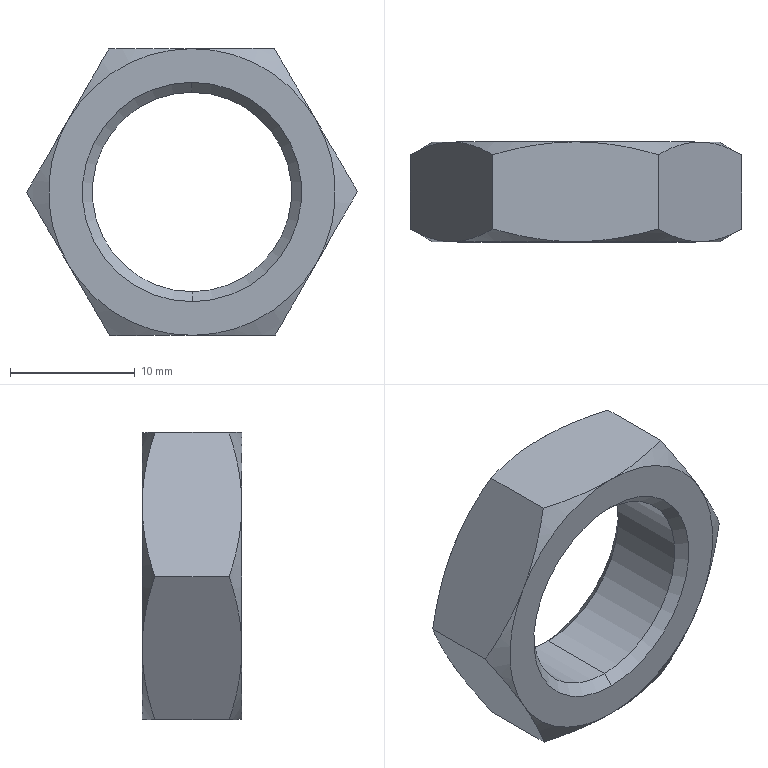Component | SolidWorks | NewCurveBenderSC63x40Cylinder-DoubleWheel-1_NewTypeCurveBenderM16x1_5-Nut-DoubleWheel-2 | 1 solid | 26 faces | box 26.56 x 8 x 23.05 mm | volume 1997 mm3 | cone 16 | plane 8 | cylinder 2 | commonest cylinder face diameters 16 x2
STEP:
#1=COLOUR_RGB('',0.7922,0.8196,0.9333);
#2=FILL_AREA_STYLE_COLOUR('',#1);
#3=FILL_AREA_STYLE('',(#2));
#4=SURFACE_STYLE_FILL_AREA(#3);
#5=SURFACE_SIDE_STYLE('',(#4));
#6=SURFACE_STYLE_USAGE(.BOTH.,#5);
#7=PRESENTATION_STYLE_ASSIGNMENT((#6));
#8=CARTESIAN_POINT('',(1.967,-10.583,0.315));
#9=VERTEX_POINT('',#8);
#10=CARTESIAN_POINT('',(1.97,-10.583,-0.315));
#11=VERTEX_POINT('',#10);
#12=CARTESIAN_POINT('',(1.969,-10.583,0.));
#13=DIRECTION('',(0.,-1.,-0.));
#14=DIRECTION('',(0.003512,0.,-1.));
#15=AXIS2_PLACEMENT_3D('',#12,#13,#14);
#16=CIRCLE('',#15,0.315);
#17=EDGE_CURVE('',#9,#11,#16,.T.);
#18=ORIENTED_EDGE('',*,*,#17,.T.);
#19=CARTESIAN_POINT('',(1.97,-10.551,-0.3465));
#20=VERTEX_POINT('',#19);
#21=CARTESIAN_POINT('',(1.97,-10.551,-0.3465));
#22=DIRECTION('',(0.002484,0.7071,-0.7071));
#23=VECTOR('',#22,39.37);
#24=LINE('',#21,#23);
#25=EDGE_CURVE('',#11,#20,#24,.T.);
#26=ORIENTED_EDGE('',*,*,#25,.T.);
#27=CARTESIAN_POINT('',(1.967,-10.551,0.3465));
#28=VERTEX_POINT('',#27);
#29=CARTESIAN_POINT('',(1.969,-10.551,0.));
#30=DIRECTION('',(0.,-1.,-0.));
#31=DIRECTION('',(0.003512,0.,-1.));
#32=AXIS2_PLACEMENT_3D('',#29,#30,#31);
#33=CIRCLE('',#32,0.3465);
#34=EDGE_CURVE('',#28,#20,#33,.T.);
#35=ORIENTED_EDGE('',*,*,#34,.F.);
#36=CARTESIAN_POINT('',(1.967,-10.551,0.3465));
#37=DIRECTION('',(-0.002484,0.7071,0.7071));
#38=VECTOR('',#37,39.37);
#39=LINE('',#36,#38);
#40=EDGE_CURVE('',#9,#28,#39,.T.);
#41=ORIENTED_EDGE('',*,*,#40,.F.);
#42=EDGE_LOOP('',(#18,#26,#35,#41));
#43=FACE_OUTER_BOUND('',#42,.T.);
#44=CARTESIAN_POINT('',(1.969,-10.551,0.));
#45=DIRECTION('',(-0.,1.,0.));
#46=DIRECTION('',(-0.003512,0.,1.));
#47=AXIS2_PLACEMENT_3D('',#44,#45,#46);
#48=CONICAL_SURFACE('',#47,0.3465,0.7854);
#49=ADVANCED_FACE('',(#43),#48,.F.);
#50=ORIENTED_EDGE('',*,*,#17,.F.);
#51=CARTESIAN_POINT('',(1.967,-10.835,0.315));
#52=VERTEX_POINT('',#51);
#53=CARTESIAN_POINT('',(1.967,-10.551,0.315));
#54=DIRECTION('',(0.,-1.,-0.));
#55=VECTOR('',#54,39.37);
#56=LINE('',#53,#55);
#57=EDGE_CURVE('',#9,#52,#56,.T.);
#58=ORIENTED_EDGE('',*,*,#57,.T.);
#59=CARTESIAN_POINT('',(1.97,-10.835,-0.315));
#60=VERTEX_POINT('',#59);
#61=CARTESIAN_POINT('',(1.969,-10.835,0.));
#62=DIRECTION('',(0.,-1.,-0.));
#63=DIRECTION('',(0.003512,0.,-1.));
#64=AXIS2_PLACEMENT_3D('',#61,#62,#63);
#65=CIRCLE('',#64,0.315);
#66=EDGE_CURVE('',#52,#60,#65,.T.);
#67=ORIENTED_EDGE('',*,*,#66,.T.);
#68=CARTESIAN_POINT('',(1.97,-10.551,-0.315));
#69=DIRECTION('',(0.,-1.,-0.));
#70=VECTOR('',#69,39.37);
#71=LINE('',#68,#70);
#72=EDGE_CURVE('',#11,#60,#71,.T.);
#73=ORIENTED_EDGE('',*,*,#72,.F.);
#74=EDGE_LOOP('',(#50,#58,#67,#73));
#75=FACE_OUTER_BOUND('',#74,.T.);
#76=CARTESIAN_POINT('',(1.969,-10.551,0.));
#77=DIRECTION('',(0.,-1.,-0.));
#78=DIRECTION('',(0.003512,0.,-1.));
#79=AXIS2_PLACEMENT_3D('',#76,#77,#78);
#80=CYLINDRICAL_SURFACE('',#79,0.315);
#81=ADVANCED_FACE('',(#75),#80,.F.);
#82=ORIENTED_EDGE('',*,*,#66,.F.);
#83=CARTESIAN_POINT('',(1.967,-10.866,0.3465));
#84=VERTEX_POINT('',#83);
#85=CARTESIAN_POINT('',(1.967,-10.835,0.315));
#86=DIRECTION('',(-0.002484,-0.7071,0.7071));
#87=VECTOR('',#86,39.37);
#88=LINE('',#85,#87);
#89=EDGE_CURVE('',#52,#84,#88,.T.);
#90=ORIENTED_EDGE('',*,*,#89,.T.);
#91=CARTESIAN_POINT('',(1.97,-10.866,-0.3465));
#92=VERTEX_POINT('',#91);
#93=CARTESIAN_POINT('',(1.969,-10.866,0.));
#94=DIRECTION('',(0.,-1.,-0.));
#95=DIRECTION('',(0.003512,0.,-1.));
#96=AXIS2_PLACEMENT_3D('',#93,#94,#95);
#97=CIRCLE('',#96,0.3465);
#98=EDGE_CURVE('',#84,#92,#97,.T.);
#99=ORIENTED_EDGE('',*,*,#98,.T.);
#100=CARTESIAN_POINT('',(1.97,-10.835,-0.315));
#101=DIRECTION('',(0.002484,-0.7071,-0.7071));
#102=VECTOR('',#101,39.37);
#103=LINE('',#100,#102);
#104=EDGE_CURVE('',#60,#92,#103,.T.);
#105=ORIENTED_EDGE('',*,*,#104,.F.);
#106=EDGE_LOOP('',(#82,#90,#99,#105));
#107=FACE_OUTER_BOUND('',#106,.T.);
#108=CARTESIAN_POINT('',(1.969,-10.835,0.));
#109=DIRECTION('',(0.,-1.,-0.));
#110=DIRECTION('',(0.003512,0.,-1.));
#111=AXIS2_PLACEMENT_3D('',#108,#109,#110);
#112=CONICAL_SURFACE('',#111,0.315,0.7854);
#113=ADVANCED_FACE('',(#107),#112,.F.);
#114=CARTESIAN_POINT('',(1.967,-10.866,0.4528));
#115=VERTEX_POINT('',#114);
#116=CARTESIAN_POINT('',(1.706,-10.826,0.4518));
#117=VERTEX_POINT('',#116);
#118=CARTESIAN_POINT('',(1.967,-10.866,0.4528));
#119=CARTESIAN_POINT('',(1.923,-10.866,0.4526));
#120=CARTESIAN_POINT('',(1.879,-10.862,0.4524));
#121=CARTESIAN_POINT('',(1.792,-10.848,0.4521));
#122=CARTESIAN_POINT('',(1.748,-10.838,0.452));
#123=CARTESIAN_POINT('',(1.706,-10.826,0.4518));
#124=B_SPLINE_CURVE_WITH_KNOTS('',3,(#118,#119,#120,#121,#122,#123),.UNSPECIFIED.,.F.,.F.,(4,2,4),(0.03588,0.03924,0.0426),.UNSPECIFIED.);
#125=EDGE_CURVE('',#115,#117,#124,.T.);
#126=ORIENTED_EDGE('',*,*,#125,.T.);
#127=CARTESIAN_POINT('',(1.576,-10.866,0.225));
#128=VERTEX_POINT('',#127);
#129=CARTESIAN_POINT('',(1.706,-10.826,0.4518));
#130=CARTESIAN_POINT('',(1.684,-10.838,0.4147));
#131=CARTESIAN_POINT('',(1.663,-10.848,0.3773));
#132=CARTESIAN_POINT('',(1.62,-10.862,0.3018));
#133=CARTESIAN_POINT('',(1.598,-10.866,0.2636));
#134=CARTESIAN_POINT('',(1.576,-10.866,0.225));
#135=B_SPLINE_CURVE_WITH_KNOTS('',3,(#129,#130,#131,#132,#133,#134),.UNSPECIFIED.,.F.,.F.,(4,2,4),(0.00000024,0.003359,0.006718),.UNSPECIFIED.);
#136=EDGE_CURVE('',#117,#128,#135,.T.);
#137=ORIENTED_EDGE('',*,*,#136,.T.);
#138=CARTESIAN_POINT('',(1.969,-10.866,0.));
#139=DIRECTION('',(0.,-1.,-0.));
#140=DIRECTION('',(0.003512,0.,-1.));
#141=AXIS2_PLACEMENT_3D('',#138,#139,#140);
#142=CIRCLE('',#141,0.4528);
#143=EDGE_CURVE('',#115,#128,#142,.T.);
#144=ORIENTED_EDGE('',*,*,#143,.F.);
#145=EDGE_LOOP('',(#126,#137,#144));
#146=FACE_OUTER_BOUND('',#145,.T.);
#147=CARTESIAN_POINT('',(1.969,-10.814,0.));
#148=DIRECTION('',(-0.,1.,0.));
#149=DIRECTION('',(-0.003512,0.,1.));
#150=AXIS2_PLACEMENT_3D('',#147,#148,#149);
#151=CONICAL_SURFACE('',#150,0.5433,1.047);
#152=ADVANCED_FACE('',(#146),#151,.T.);
#153=CARTESIAN_POINT('',(1.577,-10.866,-0.2278));
#154=VERTEX_POINT('',#153);
#155=CARTESIAN_POINT('',(1.969,-10.866,0.));
#156=DIRECTION('',(0.,-1.,-0.));
#157=DIRECTION('',(0.003512,0.,-1.));
#158=AXIS2_PLACEMENT_3D('',#155,#156,#157);
#159=CIRCLE('',#158,0.4528);
#160=EDGE_CURVE('',#128,#154,#159,.T.);
#161=ORIENTED_EDGE('',*,*,#160,.F.);
#162=CARTESIAN_POINT('',(1.446,-10.826,-0.001836));
#163=VERTEX_POINT('',#162);
#164=CARTESIAN_POINT('',(1.576,-10.866,0.225));
#165=CARTESIAN_POINT('',(1.565,-10.866,0.2057));
#166=CARTESIAN_POINT('',(1.554,-10.865,0.1864));
#167=CARTESIAN_POINT('',(1.532,-10.861,0.1482));
#168=CARTESIAN_POINT('',(1.521,-10.859,0.1292));
#169=CARTESIAN_POINT('',(1.488,-10.848,0.0725));
#170=CARTESIAN_POINT('',(1.467,-10.838,0.03518));
#171=CARTESIAN_POINT('',(1.446,-10.826,-0.001836));
#172=B_SPLINE_CURVE_WITH_KNOTS('',3,(#164,#165,#166,#167,#168,#169,#170,#171),.UNSPECIFIED.,.F.,.F.,(4,2,2,4),(0.006718,0.008392,0.01006,0.01341),.UNSPECIFIED.);
#173=EDGE_CURVE('',#128,#163,#172,.T.);
#174=ORIENTED_EDGE('',*,*,#173,.T.);
#175=CARTESIAN_POINT('',(1.446,-10.826,-0.001836));
#176=CARTESIAN_POINT('',(1.467,-10.838,-0.03879));
#177=CARTESIAN_POINT('',(1.489,-10.848,-0.07602));
#178=CARTESIAN_POINT('',(1.533,-10.862,-0.1513));
#179=CARTESIAN_POINT('',(1.555,-10.866,-0.1893));
#180=CARTESIAN_POINT('',(1.577,-10.866,-0.2278));
#181=B_SPLINE_CURVE_WITH_KNOTS('',3,(#175,#176,#177,#178,#179,#180),.UNSPECIFIED.,.F.,.F.,(4,2,4),(0.00000024,0.003359,0.006718),.UNSPECIFIED.);
#182=EDGE_CURVE('',#163,#154,#181,.T.);
#183=ORIENTED_EDGE('',*,*,#182,.T.);
#184=EDGE_LOOP('',(#161,#174,#183));
#185=FACE_OUTER_BOUND('',#184,.T.);
#186=CARTESIAN_POINT('',(1.969,-10.814,0.));
#187=DIRECTION('',(-0.,1.,0.));
#188=DIRECTION('',(-0.003512,0.,1.));
#189=AXIS2_PLACEMENT_3D('',#186,#187,#188);
#190=CONICAL_SURFACE('',#189,0.5433,1.047);
#191=ADVANCED_FACE('',(#185),#190,.T.);
#192=CARTESIAN_POINT('',(1.97,-10.866,-0.4528));
#193=VERTEX_POINT('',#192);
#194=CARTESIAN_POINT('',(1.969,-10.866,0.));
#195=DIRECTION('',(0.,-1.,-0.));
#196=DIRECTION('',(0.003512,0.,-1.));
#197=AXIS2_PLACEMENT_3D('',#194,#195,#196);
#198=CIRCLE('',#197,0.4528);
#199=EDGE_CURVE('',#154,#193,#198,.T.);
#200=ORIENTED_EDGE('',*,*,#199,.F.);
#201=CARTESIAN_POINT('',(1.709,-10.826,-0.4537));
#202=VERTEX_POINT('',#201);
#203=CARTESIAN_POINT('',(1.577,-10.866,-0.2278));
#204=CARTESIAN_POINT('',(1.588,-10.866,-0.2469));
#205=CARTESIAN_POINT('',(1.6,-10.865,-0.2662));
#206=CARTESIAN_POINT('',(1.622,-10.861,-0.3043));
#207=CARTESIAN_POINT('',(1.633,-10.859,-0.3232));
#208=CARTESIAN_POINT('',(1.666,-10.848,-0.3796));
#209=CARTESIAN_POINT('',(1.687,-10.838,-0.4168));
#210=CARTESIAN_POINT('',(1.709,-10.826,-0.4537));
#211=B_SPLINE_CURVE_WITH_KNOTS('',3,(#203,#204,#205,#206,#207,#208,#209,#210),.UNSPECIFIED.,.F.,.F.,(4,2,2,4),(0.006718,0.008392,0.01006,0.01341),.UNSPECIFIED.);
#212=EDGE_CURVE('',#154,#202,#211,.T.);
#213=ORIENTED_EDGE('',*,*,#212,.T.);
#214=CARTESIAN_POINT('',(1.709,-10.826,-0.4537));
#215=CARTESIAN_POINT('',(1.751,-10.838,-0.4535));
#216=CARTESIAN_POINT('',(1.795,-10.848,-0.4534));
#217=CARTESIAN_POINT('',(1.882,-10.862,-0.4531));
#218=CARTESIAN_POINT('',(1.926,-10.866,-0.4529));
#219=CARTESIAN_POINT('',(1.97,-10.866,-0.4528));
#220=B_SPLINE_CURVE_WITH_KNOTS('',3,(#214,#215,#216,#217,#218,#219),.UNSPECIFIED.,.F.,.F.,(4,2,4),(0.01189,0.01525,0.01861),.UNSPECIFIED.);
#221=EDGE_CURVE('',#202,#193,#220,.T.);
#222=ORIENTED_EDGE('',*,*,#221,.T.);
#223=EDGE_LOOP('',(#200,#213,#222));
#224=FACE_OUTER_BOUND('',#223,.T.);
#225=CARTESIAN_POINT('',(1.969,-10.814,0.));
#226=DIRECTION('',(-0.,1.,0.));
#227=DIRECTION('',(-0.003512,0.,1.));
#228=AXIS2_PLACEMENT_3D('',#225,#226,#227);
#229=CONICAL_SURFACE('',#228,0.5433,1.047);
#230=ADVANCED_FACE('',(#224),#229,.T.);
#231=CARTESIAN_POINT('',(2.36,-10.866,0.2278));
#232=VERTEX_POINT('',#231);
#233=CARTESIAN_POINT('',(2.228,-10.826,0.4537));
#234=VERTEX_POINT('',#233);
#235=CARTESIAN_POINT('',(2.36,-10.866,0.2278));
#236=CARTESIAN_POINT('',(2.349,-10.866,0.2469));
#237=CARTESIAN_POINT('',(2.337,-10.865,0.2662));
#238=CARTESIAN_POINT('',(2.315,-10.861,0.3043));
#239=CARTESIAN_POINT('',(2.304,-10.859,0.3232));
#240=CARTESIAN_POINT('',(2.271,-10.848,0.3796));
#241=CARTESIAN_POINT('',(2.25,-10.838,0.4168));
#242=CARTESIAN_POINT('',(2.228,-10.826,0.4537));
#243=B_SPLINE_CURVE_WITH_KNOTS('',3,(#235,#236,#237,#238,#239,#240,#241,#242),.UNSPECIFIED.,.F.,.F.,(4,2,2,4),(0.006718,0.008392,0.01006,0.01341),.UNSPECIFIED.);
#244=EDGE_CURVE('',#232,#234,#243,.T.);
#245=ORIENTED_EDGE('',*,*,#244,.T.);
#246=CARTESIAN_POINT('',(2.228,-10.826,0.4537));
#247=CARTESIAN_POINT('',(2.186,-10.838,0.4535));
#248=CARTESIAN_POINT('',(2.143,-10.848,0.4534));
#249=CARTESIAN_POINT('',(2.078,-10.859,0.4531));
#250=CARTESIAN_POINT('',(2.056,-10.861,0.4531));
#251=CARTESIAN_POINT('',(2.011,-10.865,0.4529));
#252=CARTESIAN_POINT('',(1.989,-10.866,0.4528));
#253=CARTESIAN_POINT('',(1.967,-10.866,0.4528));
#254=B_SPLINE_CURVE_WITH_KNOTS('',3,(#246,#247,#248,#249,#250,#251,#252,#253),.UNSPECIFIED.,.F.,.F.,(4,2,2,4),(0.02915,0.03251,0.03419,0.03588),.UNSPECIFIED.);
#255=EDGE_CURVE('',#234,#115,#254,.T.);
#256=ORIENTED_EDGE('',*,*,#255,.T.);
#257=CARTESIAN_POINT('',(1.969,-10.866,0.));
#258=DIRECTION('',(0.,-1.,-0.));
#259=DIRECTION('',(0.003512,0.,-1.));
#260=AXIS2_PLACEMENT_3D('',#257,#258,#259);
#261=CIRCLE('',#260,0.4528);
#262=EDGE_CURVE('',#232,#115,#261,.T.);
#263=ORIENTED_EDGE('',*,*,#262,.F.);
#264=EDGE_LOOP('',(#245,#256,#263));
#265=FACE_OUTER_BOUND('',#264,.T.);
#266=CARTESIAN_POINT('',(1.969,-10.814,0.));
#267=DIRECTION('',(-0.,1.,0.));
#268=DIRECTION('',(-0.003512,0.,1.));
#269=AXIS2_PLACEMENT_3D('',#266,#267,#268);
#270=CONICAL_SURFACE('',#269,0.5433,1.047);
#271=ADVANCED_FACE('',(#265),#270,.T.);
#272=CARTESIAN_POINT('',(2.361,-10.866,-0.225));
#273=VERTEX_POINT('',#272);
#274=CARTESIAN_POINT('',(1.969,-10.866,0.));
#275=DIRECTION('',(0.,-1.,-0.));
#276=DIRECTION('',(0.003512,0.,-1.));
#277=AXIS2_PLACEMENT_3D('',#274,#275,#276);
#278=CIRCLE('',#277,0.4528);
#279=EDGE_CURVE('',#193,#273,#278,.T.);
#280=ORIENTED_EDGE('',*,*,#279,.F.);
#281=CARTESIAN_POINT('',(2.231,-10.826,-0.4518));
#282=VERTEX_POINT('',#281);
#283=CARTESIAN_POINT('',(1.97,-10.866,-0.4528));
#284=CARTESIAN_POINT('',(1.992,-10.866,-0.4527));
#285=CARTESIAN_POINT('',(2.014,-10.865,-0.4526));
#286=CARTESIAN_POINT('',(2.059,-10.861,-0.4524));
#287=CARTESIAN_POINT('',(2.081,-10.859,-0.4524));
#288=CARTESIAN_POINT('',(2.146,-10.848,-0.4521));
#289=CARTESIAN_POINT('',(2.189,-10.838,-0.452));
#290=CARTESIAN_POINT('',(2.231,-10.826,-0.4518));
#291=B_SPLINE_CURVE_WITH_KNOTS('',3,(#283,#284,#285,#286,#287,#288,#289,#290),.UNSPECIFIED.,.F.,.F.,(4,2,2,4),(0.01861,0.02029,0.02197,0.02533),.UNSPECIFIED.);
#292=EDGE_CURVE('',#193,#282,#291,.T.);
#293=ORIENTED_EDGE('',*,*,#292,.T.);
#294=CARTESIAN_POINT('',(2.231,-10.826,-0.4518));
#295=CARTESIAN_POINT('',(2.253,-10.838,-0.4147));
#296=CARTESIAN_POINT('',(2.274,-10.848,-0.3773));
#297=CARTESIAN_POINT('',(2.317,-10.862,-0.3018));
#298=CARTESIAN_POINT('',(2.339,-10.866,-0.2636));
#299=CARTESIAN_POINT('',(2.361,-10.866,-0.225));
#300=B_SPLINE_CURVE_WITH_KNOTS('',3,(#294,#295,#296,#297,#298,#299),.UNSPECIFIED.,.F.,.F.,(4,2,4),(0.00000024,0.003359,0.006718),.UNSPECIFIED.);
#301=EDGE_CURVE('',#282,#273,#300,.T.);
#302=ORIENTED_EDGE('',*,*,#301,.T.);
#303=EDGE_LOOP('',(#280,#293,#302));
#304=FACE_OUTER_BOUND('',#303,.T.);
#305=CARTESIAN_POINT('',(1.969,-10.814,0.));
#306=DIRECTION('',(-0.,1.,0.));
#307=DIRECTION('',(-0.003512,0.,1.));
#308=AXIS2_PLACEMENT_3D('',#305,#306,#307);
#309=CONICAL_SURFACE('',#308,0.5433,1.047);
#310=ADVANCED_FACE('',(#304),#309,.T.);
#311=CARTESIAN_POINT('',(1.969,-10.866,0.));
#312=DIRECTION('',(0.,-1.,-0.));
#313=DIRECTION('',(0.003512,0.,-1.));
#314=AXIS2_PLACEMENT_3D('',#311,#312,#313);
#315=CIRCLE('',#314,0.3465);
#316=EDGE_CURVE('',#92,#84,#315,.T.);
#317=ORIENTED_EDGE('',*,*,#316,.F.);
#318=ORIENTED_EDGE('',*,*,#98,.F.);
#319=EDGE_LOOP('',(#317,#318));
#320=FACE_BOUND('',#319,.T.);
#321=ORIENTED_EDGE('',*,*,#279,.T.);
#322=CARTESIAN_POINT('',(1.969,-10.866,0.));
#323=DIRECTION('',(0.,-1.,-0.));
#324=DIRECTION('',(0.003512,0.,-1.));
#325=AXIS2_PLACEMENT_3D('',#322,#323,#324);
#326=CIRCLE('',#325,0.4528);
#327=EDGE_CURVE('',#273,#232,#326,.T.);
#328=ORIENTED_EDGE('',*,*,#327,.T.);
#329=ORIENTED_EDGE('',*,*,#262,.T.);
#330=ORIENTED_EDGE('',*,*,#143,.T.);
#331=ORIENTED_EDGE('',*,*,#160,.T.);
#332=ORIENTED_EDGE('',*,*,#199,.T.);
#333=EDGE_LOOP('',(#321,#328,#329,#330,#331,#332));
#334=FACE_OUTER_BOUND('',#333,.T.);
#335=CARTESIAN_POINT('',(1.969,-10.866,0.));
#336=DIRECTION('',(-0.,1.,0.));
#337=DIRECTION('',(-0.003512,-0.,1.));
#338=AXIS2_PLACEMENT_3D('',#335,#336,#337);
#339=PLANE('',#338);
#340=ADVANCED_FACE('',(#320,#334),#339,.F.);
#341=CARTESIAN_POINT('',(2.491,-10.826,0.001836));
#342=VERTEX_POINT('',#341);
#343=CARTESIAN_POINT('',(2.361,-10.866,-0.225));
#344=CARTESIAN_POINT('',(2.372,-10.866,-0.2057));
#345=CARTESIAN_POINT('',(2.383,-10.865,-0.1864));
#346=CARTESIAN_POINT('',(2.405,-10.861,-0.1482));
#347=CARTESIAN_POINT('',(2.416,-10.859,-0.1292));
#348=CARTESIAN_POINT('',(2.449,-10.848,-0.0725));
#349=CARTESIAN_POINT('',(2.47,-10.838,-0.03518));
#350=CARTESIAN_POINT('',(2.491,-10.826,0.001836));
#351=B_SPLINE_CURVE_WITH_KNOTS('',3,(#343,#344,#345,#346,#347,#348,#349,#350),.UNSPECIFIED.,.F.,.F.,(4,2,2,4),(0.006718,0.008392,0.01006,0.01341),.UNSPECIFIED.);
#352=EDGE_CURVE('',#273,#342,#351,.T.);
#353=ORIENTED_EDGE('',*,*,#352,.T.);
#354=CARTESIAN_POINT('',(2.491,-10.826,0.001836));
#355=CARTESIAN_POINT('',(2.47,-10.838,0.03879));
#356=CARTESIAN_POINT('',(2.448,-10.848,0.07602));
#357=CARTESIAN_POINT('',(2.404,-10.862,0.1513));
#358=CARTESIAN_POINT('',(2.382,-10.866,0.1893));
#359=CARTESIAN_POINT('',(2.36,-10.866,0.2278));
#360=B_SPLINE_CURVE_WITH_KNOTS('',3,(#354,#355,#356,#357,#358,#359),.UNSPECIFIED.,.F.,.F.,(4,2,4),(0.00000024,0.003359,0.006718),.UNSPECIFIED.);
#361=EDGE_CURVE('',#342,#232,#360,.T.);
#362=ORIENTED_EDGE('',*,*,#361,.T.);
#363=ORIENTED_EDGE('',*,*,#327,.F.);
#364=EDGE_LOOP('',(#353,#362,#363));
#365=FACE_OUTER_BOUND('',#364,.T.);
#366=CARTESIAN_POINT('',(1.969,-10.814,0.));
#367=DIRECTION('',(-0.,1.,0.));
#368=DIRECTION('',(-0.003512,0.,1.));
#369=AXIS2_PLACEMENT_3D('',#366,#367,#368);
#370=CONICAL_SURFACE('',#369,0.5433,1.047);
#371=ADVANCED_FACE('',(#365),#370,.T.);
#372=CARTESIAN_POINT('',(1.709,-10.592,-0.4537));
#373=VERTEX_POINT('',#372);
#374=CARTESIAN_POINT('',(1.709,-10.236,-0.4537));
#375=DIRECTION('',(0.,-1.,-0.));
#376=VECTOR('',#375,39.37);
#377=LINE('',#374,#376);
#378=EDGE_CURVE('',#373,#202,#377,.T.);
#379=ORIENTED_EDGE('',*,*,#378,.F.);
#380=CARTESIAN_POINT('',(1.97,-10.551,-0.4528));
#381=VERTEX_POINT('',#380);
#382=CARTESIAN_POINT('',(1.97,-10.551,-0.4528));
#383=CARTESIAN_POINT('',(1.926,-10.551,-0.4529));
#384=CARTESIAN_POINT('',(1.882,-10.555,-0.4531));
#385=CARTESIAN_POINT('',(1.795,-10.569,-0.4534));
#386=CARTESIAN_POINT('',(1.751,-10.579,-0.4535));
#387=CARTESIAN_POINT('',(1.709,-10.592,-0.4537));
#388=B_SPLINE_CURVE_WITH_KNOTS('',3,(#382,#383,#384,#385,#386,#387),.UNSPECIFIED.,.F.,.F.,(4,2,4),(0.03588,0.03924,0.0426),.UNSPECIFIED.);
#389=EDGE_CURVE('',#381,#373,#388,.T.);
#390=ORIENTED_EDGE('',*,*,#389,.F.);
#391=CARTESIAN_POINT('',(2.231,-10.592,-0.4518));
#392=VERTEX_POINT('',#391);
#393=CARTESIAN_POINT('',(2.231,-10.592,-0.4518));
#394=CARTESIAN_POINT('',(2.189,-10.579,-0.452));
#395=CARTESIAN_POINT('',(2.146,-10.569,-0.4521));
#396=CARTESIAN_POINT('',(2.081,-10.559,-0.4524));
#397=CARTESIAN_POINT('',(2.059,-10.556,-0.4524));
#398=CARTESIAN_POINT('',(2.014,-10.552,-0.4526));
#399=CARTESIAN_POINT('',(1.992,-10.551,-0.4527));
#400=CARTESIAN_POINT('',(1.97,-10.551,-0.4528));
#401=B_SPLINE_CURVE_WITH_KNOTS('',3,(#393,#394,#395,#396,#397,#398,#399,#400),.UNSPECIFIED.,.F.,.F.,(4,2,2,4),(0.02915,0.03251,0.03419,0.03588),.UNSPECIFIED.);
#402=EDGE_CURVE('',#392,#381,#401,.T.);
#403=ORIENTED_EDGE('',*,*,#402,.F.);
#404=CARTESIAN_POINT('',(2.231,-10.236,-0.4518));
#405=DIRECTION('',(0.,-1.,-0.));
#406=VECTOR('',#405,39.37);
#407=LINE('',#404,#406);
#408=EDGE_CURVE('',#392,#282,#407,.T.);
#409=ORIENTED_EDGE('',*,*,#408,.T.);
#410=ORIENTED_EDGE('',*,*,#292,.F.);
#411=ORIENTED_EDGE('',*,*,#221,.F.);
#412=EDGE_LOOP('',(#379,#390,#403,#409,#410,#411));
#413=FACE_OUTER_BOUND('',#412,.T.);
#414=CARTESIAN_POINT('',(2.231,-10.236,-0.4518));
#415=DIRECTION('',(-0.003512,-0.,1.));
#416=DIRECTION('',(0.,-1.,-0.));
#417=AXIS2_PLACEMENT_3D('',#414,#415,#416);
#418=PLANE('',#417);
#419=ADVANCED_FACE('',(#413),#418,.F.);
#420=CARTESIAN_POINT('',(1.446,-10.592,-0.001836));
#421=VERTEX_POINT('',#420);
#422=CARTESIAN_POINT('',(1.446,-10.236,-0.001836));
#423=DIRECTION('',(0.,-1.,-0.));
#424=VECTOR('',#423,39.37);
#425=LINE('',#422,#424);
#426=EDGE_CURVE('',#421,#163,#425,.T.);
#427=ORIENTED_EDGE('',*,*,#426,.F.);
#428=CARTESIAN_POINT('',(1.577,-10.551,-0.2278));
#429=VERTEX_POINT('',#428);
#430=CARTESIAN_POINT('',(1.577,-10.551,-0.2278));
#431=CARTESIAN_POINT('',(1.566,-10.551,-0.2086));
#432=CARTESIAN_POINT('',(1.555,-10.552,-0.1893));
#433=CARTESIAN_POINT('',(1.533,-10.556,-0.1512));
#434=CARTESIAN_POINT('',(1.522,-10.559,-0.1323));
#435=CARTESIAN_POINT('',(1.489,-10.569,-0.07587));
#436=CARTESIAN_POINT('',(1.467,-10.579,-0.0387));
#437=CARTESIAN_POINT('',(1.446,-10.592,-0.001836));
#438=B_SPLINE_CURVE_WITH_KNOTS('',3,(#430,#431,#432,#433,#434,#435,#436,#437),.UNSPECIFIED.,.F.,.F.,(4,2,2,4),(0.006718,0.008392,0.01006,0.01341),.UNSPECIFIED.);
#439=EDGE_CURVE('',#429,#421,#438,.T.);
#440=ORIENTED_EDGE('',*,*,#439,.F.);
#441=CARTESIAN_POINT('',(1.709,-10.592,-0.4537));
#442=CARTESIAN_POINT('',(1.687,-10.579,-0.4167));
#443=CARTESIAN_POINT('',(1.666,-10.569,-0.3795));
#444=CARTESIAN_POINT('',(1.622,-10.555,-0.3043));
#445=CARTESIAN_POINT('',(1.6,-10.551,-0.2662));
#446=CARTESIAN_POINT('',(1.577,-10.551,-0.2278));
#447=B_SPLINE_CURVE_WITH_KNOTS('',3,(#441,#442,#443,#444,#445,#446),.UNSPECIFIED.,.F.,.F.,(4,2,4),(0.00000024,0.003359,0.006718),.UNSPECIFIED.);
#448=EDGE_CURVE('',#373,#429,#447,.T.);
#449=ORIENTED_EDGE('',*,*,#448,.F.);
#450=ORIENTED_EDGE('',*,*,#378,.T.);
#451=ORIENTED_EDGE('',*,*,#212,.F.);
#452=ORIENTED_EDGE('',*,*,#182,.F.);
#453=EDGE_LOOP('',(#427,#440,#449,#450,#451,#452));
#454=FACE_OUTER_BOUND('',#453,.T.);
#455=CARTESIAN_POINT('',(1.709,-10.236,-0.4537));
#456=DIRECTION('',(0.8643,0.,0.503));
#457=DIRECTION('',(0.503,0.,-0.8643));
#458=AXIS2_PLACEMENT_3D('',#455,#456,#457);
#459=PLANE('',#458);
#460=ADVANCED_FACE('',(#454),#459,.F.);
#461=CARTESIAN_POINT('',(1.706,-10.592,0.4518));
#462=VERTEX_POINT('',#461);
#463=CARTESIAN_POINT('',(1.706,-10.236,0.4518));
#464=DIRECTION('',(0.,-1.,-0.));
#465=VECTOR('',#464,39.37);
#466=LINE('',#463,#465);
#467=EDGE_CURVE('',#462,#117,#466,.T.);
#468=ORIENTED_EDGE('',*,*,#467,.F.);
#469=CARTESIAN_POINT('',(1.576,-10.551,0.225));
#470=VERTEX_POINT('',#469);
#471=CARTESIAN_POINT('',(1.576,-10.551,0.225));
#472=CARTESIAN_POINT('',(1.587,-10.551,0.2443));
#473=CARTESIAN_POINT('',(1.598,-10.552,0.2636));
#474=CARTESIAN_POINT('',(1.62,-10.556,0.3018));
#475=CARTESIAN_POINT('',(1.63,-10.559,0.3208));
#476=CARTESIAN_POINT('',(1.663,-10.569,0.3775));
#477=CARTESIAN_POINT('',(1.684,-10.579,0.4148));
#478=CARTESIAN_POINT('',(1.706,-10.592,0.4518));
#479=B_SPLINE_CURVE_WITH_KNOTS('',3,(#471,#472,#473,#474,#475,#476,#477,#478),.UNSPECIFIED.,.F.,.F.,(4,2,2,4),(0.006718,0.008392,0.01006,0.01341),.UNSPECIFIED.);
#480=EDGE_CURVE('',#470,#462,#479,.T.);
#481=ORIENTED_EDGE('',*,*,#480,.F.);
#482=CARTESIAN_POINT('',(1.446,-10.592,-0.001836));
#483=CARTESIAN_POINT('',(1.467,-10.579,0.03527));
#484=CARTESIAN_POINT('',(1.488,-10.569,0.07265));
#485=CARTESIAN_POINT('',(1.532,-10.555,0.1482));
#486=CARTESIAN_POINT('',(1.553,-10.551,0.1864));
#487=CARTESIAN_POINT('',(1.576,-10.551,0.225));
#488=B_SPLINE_CURVE_WITH_KNOTS('',3,(#482,#483,#484,#485,#486,#487),.UNSPECIFIED.,.F.,.F.,(4,2,4),(0.00000024,0.003359,0.006718),.UNSPECIFIED.);
#489=EDGE_CURVE('',#421,#470,#488,.T.);
#490=ORIENTED_EDGE('',*,*,#489,.F.);
#491=ORIENTED_EDGE('',*,*,#426,.T.);
#492=ORIENTED_EDGE('',*,*,#173,.F.);
#493=ORIENTED_EDGE('',*,*,#136,.F.);
#494=EDGE_LOOP('',(#468,#481,#490,#491,#492,#493));
#495=FACE_OUTER_BOUND('',#494,.T.);
#496=CARTESIAN_POINT('',(1.446,-10.236,-0.001836));
#497=DIRECTION('',(0.8678,0.,-0.497));
#498=DIRECTION('',(-0.497,-0.,-0.8678));
#499=AXIS2_PLACEMENT_3D('',#496,#497,#498);
#500=PLANE('',#499);
#501=ADVANCED_FACE('',(#495),#500,.F.);
#502=CARTESIAN_POINT('',(2.228,-10.592,0.4537));
#503=VERTEX_POINT('',#502);
#504=CARTESIAN_POINT('',(2.228,-10.236,0.4537));
#505=DIRECTION('',(0.,-1.,-0.));
#506=VECTOR('',#505,39.37);
#507=LINE('',#504,#506);
#508=EDGE_CURVE('',#503,#234,#507,.T.);
#509=ORIENTED_EDGE('',*,*,#508,.F.);
#510=CARTESIAN_POINT('',(1.967,-10.551,0.4528));
#511=VERTEX_POINT('',#510);
#512=CARTESIAN_POINT('',(1.967,-10.551,0.4528));
#513=CARTESIAN_POINT('',(1.989,-10.551,0.4528));
#514=CARTESIAN_POINT('',(2.011,-10.552,0.4529));
#515=CARTESIAN_POINT('',(2.056,-10.556,0.4531));
#516=CARTESIAN_POINT('',(2.078,-10.559,0.4531));
#517=CARTESIAN_POINT('',(2.143,-10.569,0.4534));
#518=CARTESIAN_POINT('',(2.186,-10.579,0.4535));
#519=CARTESIAN_POINT('',(2.228,-10.592,0.4537));
#520=B_SPLINE_CURVE_WITH_KNOTS('',3,(#512,#513,#514,#515,#516,#517,#518,#519),.UNSPECIFIED.,.F.,.F.,(4,2,2,4),(0.01861,0.02029,0.02197,0.02533),.UNSPECIFIED.);
#521=EDGE_CURVE('',#511,#503,#520,.T.);
#522=ORIENTED_EDGE('',*,*,#521,.F.);
#523=CARTESIAN_POINT('',(1.706,-10.592,0.4518));
#524=CARTESIAN_POINT('',(1.748,-10.579,0.452));
#525=CARTESIAN_POINT('',(1.792,-10.569,0.4521));
#526=CARTESIAN_POINT('',(1.879,-10.555,0.4524));
#527=CARTESIAN_POINT('',(1.923,-10.551,0.4526));
#528=CARTESIAN_POINT('',(1.967,-10.551,0.4528));
#529=B_SPLINE_CURVE_WITH_KNOTS('',3,(#523,#524,#525,#526,#527,#528),.UNSPECIFIED.,.F.,.F.,(4,2,4),(0.01189,0.01525,0.01861),.UNSPECIFIED.);
#530=EDGE_CURVE('',#462,#511,#529,.T.);
#531=ORIENTED_EDGE('',*,*,#530,.F.);
#532=ORIENTED_EDGE('',*,*,#467,.T.);
#533=ORIENTED_EDGE('',*,*,#125,.F.);
#534=ORIENTED_EDGE('',*,*,#255,.F.);
#535=EDGE_LOOP('',(#509,#522,#531,#532,#533,#534));
#536=FACE_OUTER_BOUND('',#535,.T.);
#537=CARTESIAN_POINT('',(1.706,-10.236,0.4518));
#538=DIRECTION('',(0.003512,0.,-1.));
#539=DIRECTION('',(-0.,1.,0.));
#540=AXIS2_PLACEMENT_3D('',#537,#538,#539);
#541=PLANE('',#540);
#542=ADVANCED_FACE('',(#536),#541,.F.);
#543=CARTESIAN_POINT('',(2.491,-10.592,0.001836));
#544=VERTEX_POINT('',#543);
#545=CARTESIAN_POINT('',(2.491,-10.236,0.001836));
#546=DIRECTION('',(0.,-1.,-0.));
#547=VECTOR('',#546,39.37);
#548=LINE('',#545,#547);
#549=EDGE_CURVE('',#544,#342,#548,.T.);
#550=ORIENTED_EDGE('',*,*,#549,.F.);
#551=CARTESIAN_POINT('',(2.36,-10.551,0.2278));
#552=VERTEX_POINT('',#551);
#553=CARTESIAN_POINT('',(2.36,-10.551,0.2278));
#554=CARTESIAN_POINT('',(2.371,-10.551,0.2086));
#555=CARTESIAN_POINT('',(2.382,-10.552,0.1893));
#556=CARTESIAN_POINT('',(2.404,-10.556,0.1512));
#557=CARTESIAN_POINT('',(2.415,-10.559,0.1323));
#558=CARTESIAN_POINT('',(2.448,-10.569,0.07587));
#559=CARTESIAN_POINT('',(2.47,-10.579,0.0387));
#560=CARTESIAN_POINT('',(2.491,-10.592,0.001836));
#561=B_SPLINE_CURVE_WITH_KNOTS('',3,(#553,#554,#555,#556,#557,#558,#559,#560),.UNSPECIFIED.,.F.,.F.,(4,2,2,4),(0.006718,0.008392,0.01006,0.01341),.UNSPECIFIED.);
#562=EDGE_CURVE('',#552,#544,#561,.T.);
#563=ORIENTED_EDGE('',*,*,#562,.F.);
#564=CARTESIAN_POINT('',(2.228,-10.592,0.4537));
#565=CARTESIAN_POINT('',(2.25,-10.579,0.4167));
#566=CARTESIAN_POINT('',(2.271,-10.569,0.3795));
#567=CARTESIAN_POINT('',(2.315,-10.555,0.3043));
#568=CARTESIAN_POINT('',(2.337,-10.551,0.2662));
#569=CARTESIAN_POINT('',(2.36,-10.551,0.2278));
#570=B_SPLINE_CURVE_WITH_KNOTS('',3,(#564,#565,#566,#567,#568,#569),.UNSPECIFIED.,.F.,.F.,(4,2,4),(0.00000024,0.003359,0.006718),.UNSPECIFIED.);
#571=EDGE_CURVE('',#503,#552,#570,.T.);
#572=ORIENTED_EDGE('',*,*,#571,.F.);
#573=ORIENTED_EDGE('',*,*,#508,.T.);
#574=ORIENTED_EDGE('',*,*,#244,.F.);
#575=ORIENTED_EDGE('',*,*,#361,.F.);
#576=EDGE_LOOP('',(#550,#563,#572,#573,#574,#575));
#577=FACE_OUTER_BOUND('',#576,.T.);
#578=CARTESIAN_POINT('',(2.228,-10.236,0.4537));
#579=DIRECTION('',(-0.8643,-0.,-0.503));
#580=DIRECTION('',(-0.503,-0.,0.8643));
#581=AXIS2_PLACEMENT_3D('',#578,#579,#580);
#582=PLANE('',#581);
#583=ADVANCED_FACE('',(#577),#582,.F.);
#584=ORIENTED_EDGE('',*,*,#408,.F.);
#585=CARTESIAN_POINT('',(2.361,-10.551,-0.225));
#586=VERTEX_POINT('',#585);
#587=CARTESIAN_POINT('',(2.361,-10.551,-0.225));
#588=CARTESIAN_POINT('',(2.35,-10.551,-0.2443));
#589=CARTESIAN_POINT('',(2.339,-10.552,-0.2636));
#590=CARTESIAN_POINT('',(2.317,-10.556,-0.3018));
#591=CARTESIAN_POINT('',(2.307,-10.559,-0.3208));
#592=CARTESIAN_POINT('',(2.274,-10.569,-0.3775));
#593=CARTESIAN_POINT('',(2.253,-10.579,-0.4148));
#594=CARTESIAN_POINT('',(2.231,-10.592,-0.4518));
#595=B_SPLINE_CURVE_WITH_KNOTS('',3,(#587,#588,#589,#590,#591,#592,#593,#594),.UNSPECIFIED.,.F.,.F.,(4,2,2,4),(0.006718,0.008392,0.01006,0.01341),.UNSPECIFIED.);
#596=EDGE_CURVE('',#586,#392,#595,.T.);
#597=ORIENTED_EDGE('',*,*,#596,.F.);
#598=CARTESIAN_POINT('',(2.491,-10.592,0.001836));
#599=CARTESIAN_POINT('',(2.47,-10.579,-0.03527));
#600=CARTESIAN_POINT('',(2.449,-10.569,-0.07265));
#601=CARTESIAN_POINT('',(2.405,-10.555,-0.1482));
#602=CARTESIAN_POINT('',(2.384,-10.551,-0.1864));
#603=CARTESIAN_POINT('',(2.361,-10.551,-0.225));
#604=B_SPLINE_CURVE_WITH_KNOTS('',3,(#598,#599,#600,#601,#602,#603),.UNSPECIFIED.,.F.,.F.,(4,2,4),(0.00000024,0.003359,0.006718),.UNSPECIFIED.);
#605=EDGE_CURVE('',#544,#586,#604,.T.);
#606=ORIENTED_EDGE('',*,*,#605,.F.);
#607=ORIENTED_EDGE('',*,*,#549,.T.);
#608=ORIENTED_EDGE('',*,*,#352,.F.);
#609=ORIENTED_EDGE('',*,*,#301,.F.);
#610=EDGE_LOOP('',(#584,#597,#606,#607,#608,#609));
#611=FACE_OUTER_BOUND('',#610,.T.);
#612=CARTESIAN_POINT('',(2.491,-10.236,0.001836));
#613=DIRECTION('',(-0.8678,-0.,0.497));
#614=DIRECTION('',(0.497,0.,0.8678));
#615=AXIS2_PLACEMENT_3D('',#612,#613,#614);
#616=PLANE('',#615);
#617=ADVANCED_FACE('',(#611),#616,.F.);
#618=CARTESIAN_POINT('',(1.969,-10.551,0.));
#619=DIRECTION('',(0.,-1.,-0.));
#620=DIRECTION('',(0.003512,0.,-1.));
#621=AXIS2_PLACEMENT_3D('',#618,#619,#620);
#622=CIRCLE('',#621,0.4528);
#623=EDGE_CURVE('',#586,#552,#622,.T.);
#624=ORIENTED_EDGE('',*,*,#623,.T.);
#625=ORIENTED_EDGE('',*,*,#562,.T.);
#626=ORIENTED_EDGE('',*,*,#605,.T.);
#627=EDGE_LOOP('',(#624,#625,#626));
#628=FACE_OUTER_BOUND('',#627,.T.);
#629=CARTESIAN_POINT('',(1.969,-10.551,0.));
#630=DIRECTION('',(0.,-1.,-0.));
#631=DIRECTION('',(0.003512,0.,-1.));
#632=AXIS2_PLACEMENT_3D('',#629,#630,#631);
#633=CONICAL_SURFACE('',#632,0.4528,1.047);
#634=ADVANCED_FACE('',(#628),#633,.T.);
#635=CARTESIAN_POINT('',(1.969,-10.551,0.));
#636=DIRECTION('',(0.,-1.,-0.));
#637=DIRECTION('',(0.003512,0.,-1.));
#638=AXIS2_PLACEMENT_3D('',#635,#636,#637);
#639=CIRCLE('',#638,0.4528);
#640=EDGE_CURVE('',#552,#511,#639,.T.);
#641=ORIENTED_EDGE('',*,*,#640,.T.);
#642=ORIENTED_EDGE('',*,*,#521,.T.);
#643=ORIENTED_EDGE('',*,*,#571,.T.);
#644=EDGE_LOOP('',(#641,#642,#643));
#645=FACE_OUTER_BOUND('',#644,.T.);
#646=CARTESIAN_POINT('',(1.969,-10.551,0.));
#647=DIRECTION('',(0.,-1.,-0.));
#648=DIRECTION('',(0.003512,0.,-1.));
#649=AXIS2_PLACEMENT_3D('',#646,#647,#648);
#650=CONICAL_SURFACE('',#649,0.4528,1.047);
#651=ADVANCED_FACE('',(#645),#650,.T.);
#652=CARTESIAN_POINT('',(1.969,-10.551,0.));
#653=DIRECTION('',(0.,-1.,-0.));
#654=DIRECTION('',(0.003512,0.,-1.));
#655=AXIS2_PLACEMENT_3D('',#652,#653,#654);
#656=CIRCLE('',#655,0.4528);
#657=EDGE_CURVE('',#511,#470,#656,.T.);
#658=ORIENTED_EDGE('',*,*,#657,.T.);
#659=ORIENTED_EDGE('',*,*,#480,.T.);
#660=ORIENTED_EDGE('',*,*,#530,.T.);
#661=EDGE_LOOP('',(#658,#659,#660));
#662=FACE_OUTER_BOUND('',#661,.T.);
#663=CARTESIAN_POINT('',(1.969,-10.551,0.));
#664=DIRECTION('',(0.,-1.,-0.));
#665=DIRECTION('',(0.003512,0.,-1.));
#666=AXIS2_PLACEMENT_3D('',#663,#664,#665);
#667=CONICAL_SURFACE('',#666,0.4528,1.047);
#668=ADVANCED_FACE('',(#662),#667,.T.);
#669=CARTESIAN_POINT('',(1.969,-10.551,0.));
#670=DIRECTION('',(0.,-1.,-0.));
#671=DIRECTION('',(0.003512,0.,-1.));
#672=AXIS2_PLACEMENT_3D('',#669,#670,#671);
#673=CIRCLE('',#672,0.4528);
#674=EDGE_CURVE('',#470,#429,#673,.T.);
#675=ORIENTED_EDGE('',*,*,#674,.T.);
#676=ORIENTED_EDGE('',*,*,#439,.T.);
#677=ORIENTED_EDGE('',*,*,#489,.T.);
#678=EDGE_LOOP('',(#675,#676,#677));
#679=FACE_OUTER_BOUND('',#678,.T.);
#680=CARTESIAN_POINT('',(1.969,-10.551,0.));
#681=DIRECTION('',(0.,-1.,-0.));
#682=DIRECTION('',(0.003512,0.,-1.));
#683=AXIS2_PLACEMENT_3D('',#680,#681,#682);
#684=CONICAL_SURFACE('',#683,0.4528,1.047);
#685=ADVANCED_FACE('',(#679),#684,.T.);
#686=CARTESIAN_POINT('',(1.969,-10.551,0.));
#687=DIRECTION('',(0.,-1.,-0.));
#688=DIRECTION('',(0.003512,0.,-1.));
#689=AXIS2_PLACEMENT_3D('',#686,#687,#688);
#690=CIRCLE('',#689,0.4528);
#691=EDGE_CURVE('',#429,#381,#690,.T.);
#692=ORIENTED_EDGE('',*,*,#691,.T.);
#693=ORIENTED_EDGE('',*,*,#389,.T.);
#694=ORIENTED_EDGE('',*,*,#448,.T.);
#695=EDGE_LOOP('',(#692,#693,#694));
#696=FACE_OUTER_BOUND('',#695,.T.);
#697=CARTESIAN_POINT('',(1.969,-10.551,0.));
#698=DIRECTION('',(0.,-1.,-0.));
#699=DIRECTION('',(0.003512,0.,-1.));
#700=AXIS2_PLACEMENT_3D('',#697,#698,#699);
#701=CONICAL_SURFACE('',#700,0.4528,1.047);
#702=ADVANCED_FACE('',(#696),#701,.T.);
#703=ORIENTED_EDGE('',*,*,#34,.T.);
#704=CARTESIAN_POINT('',(1.969,-10.551,0.));
#705=DIRECTION('',(0.,-1.,-0.));
#706=DIRECTION('',(0.003512,0.,-1.));
#707=AXIS2_PLACEMENT_3D('',#704,#705,#706);
#708=CIRCLE('',#707,0.3465);
#709=EDGE_CURVE('',#20,#28,#708,.T.);
#710=ORIENTED_EDGE('',*,*,#709,.T.);
#711=EDGE_LOOP('',(#703,#710));
#712=FACE_BOUND('',#711,.T.);
#713=CARTESIAN_POINT('',(1.969,-10.551,0.));
#714=DIRECTION('',(0.,-1.,-0.));
#715=DIRECTION('',(0.003512,0.,-1.));
#716=AXIS2_PLACEMENT_3D('',#713,#714,#715);
#717=CIRCLE('',#716,0.4528);
#718=EDGE_CURVE('',#381,#586,#717,.T.);
#719=ORIENTED_EDGE('',*,*,#718,.F.);
#720=ORIENTED_EDGE('',*,*,#691,.F.);
#721=ORIENTED_EDGE('',*,*,#674,.F.);
#722=ORIENTED_EDGE('',*,*,#657,.F.);
#723=ORIENTED_EDGE('',*,*,#640,.F.);
#724=ORIENTED_EDGE('',*,*,#623,.F.);
#725=EDGE_LOOP('',(#719,#720,#721,#722,#723,#724));
#726=FACE_OUTER_BOUND('',#725,.T.);
#727=CARTESIAN_POINT('',(2.421,-10.551,0.00159));
#728=DIRECTION('',(0.,-1.,-0.));
#729=DIRECTION('',(0.003512,0.,-1.));
#730=AXIS2_PLACEMENT_3D('',#727,#728,#729);
#731=PLANE('',#730);
#732=ADVANCED_FACE('',(#712,#726),#731,.F.);
#733=ORIENTED_EDGE('',*,*,#596,.T.);
#734=ORIENTED_EDGE('',*,*,#402,.T.);
#735=ORIENTED_EDGE('',*,*,#718,.T.);
#736=EDGE_LOOP('',(#733,#734,#735));
#737=FACE_OUTER_BOUND('',#736,.T.);
#738=CARTESIAN_POINT('',(1.969,-10.551,0.));
#739=DIRECTION('',(0.,-1.,-0.));
#740=DIRECTION('',(0.003512,0.,-1.));
#741=AXIS2_PLACEMENT_3D('',#738,#739,#740);
#742=CONICAL_SURFACE('',#741,0.4528,1.047);
#743=ADVANCED_FACE('',(#737),#742,.T.);
#744=ORIENTED_EDGE('',*,*,#89,.F.);
#745=CARTESIAN_POINT('',(1.969,-10.835,0.));
#746=DIRECTION('',(0.,-1.,-0.));
#747=DIRECTION('',(0.003512,0.,-1.));
#748=AXIS2_PLACEMENT_3D('',#745,#746,#747);
#749=CIRCLE('',#748,0.315);
#750=EDGE_CURVE('',#60,#52,#749,.T.);
#751=ORIENTED_EDGE('',*,*,#750,.F.);
#752=ORIENTED_EDGE('',*,*,#104,.T.);
#753=ORIENTED_EDGE('',*,*,#316,.T.);
#754=EDGE_LOOP('',(#744,#751,#752,#753));
#755=FACE_OUTER_BOUND('',#754,.T.);
#756=CARTESIAN_POINT('',(1.969,-10.835,0.));
#757=DIRECTION('',(0.,-1.,-0.));
#758=DIRECTION('',(0.003512,0.,-1.));
#759=AXIS2_PLACEMENT_3D('',#756,#757,#758);
#760=CONICAL_SURFACE('',#759,0.315,0.7854);
#761=ADVANCED_FACE('',(#755),#760,.F.);
#762=ORIENTED_EDGE('',*,*,#57,.F.);
#763=CARTESIAN_POINT('',(1.969,-10.583,0.));
#764=DIRECTION('',(0.,-1.,-0.));
#765=DIRECTION('',(0.003512,0.,-1.));
#766=AXIS2_PLACEMENT_3D('',#763,#764,#765);
#767=CIRCLE('',#766,0.315);
#768=EDGE_CURVE('',#11,#9,#767,.T.);
#769=ORIENTED_EDGE('',*,*,#768,.F.);
#770=ORIENTED_EDGE('',*,*,#72,.T.);
#771=ORIENTED_EDGE('',*,*,#750,.T.);
#772=EDGE_LOOP('',(#762,#769,#770,#771));
#773=FACE_OUTER_BOUND('',#772,.T.);
#774=CARTESIAN_POINT('',(1.969,-10.551,0.));
#775=DIRECTION('',(0.,-1.,-0.));
#776=DIRECTION('',(0.003512,0.,-1.));
#777=AXIS2_PLACEMENT_3D('',#774,#775,#776);
#778=CYLINDRICAL_SURFACE('',#777,0.315);
#779=ADVANCED_FACE('',(#773),#778,.F.);
#780=ORIENTED_EDGE('',*,*,#25,.F.);
#781=ORIENTED_EDGE('',*,*,#768,.T.);
#782=ORIENTED_EDGE('',*,*,#40,.T.);
#783=ORIENTED_EDGE('',*,*,#709,.F.);
#784=EDGE_LOOP('',(#780,#781,#782,#783));
#785=FACE_OUTER_BOUND('',#784,.T.);
#786=CARTESIAN_POINT('',(1.969,-10.551,0.));
#787=DIRECTION('',(-0.,1.,0.));
#788=DIRECTION('',(-0.003512,0.,1.));
#789=AXIS2_PLACEMENT_3D('',#786,#787,#788);
#790=CONICAL_SURFACE('',#789,0.3465,0.7854);
#791=ADVANCED_FACE('',(#785),#790,.F.);
#792=CLOSED_SHELL('',(#49,#81,#113,#152,#191,#230,#271,#310,#340,#371,#419,#460,#501,#542,#583,#617,#634,#651,#668,#685,#702,#732,#743,#761,#779,#791));
#793=MANIFOLD_SOLID_BREP('',#792);
#794=STYLED_ITEM('',(#7),#793);
#795=PRESENTATION_LAYER_ASSIGNMENT('','',(#794));
#796=(LENGTH_UNIT()NAMED_UNIT(*)SI_UNIT($,.METRE.));
#797=LENGTH_MEASURE_WITH_UNIT(LENGTH_MEASURE(0.0254),#796);
#798=DIMENSIONAL_EXPONENTS(1.,0.,0.,0.,0.,0.,0.);
#799=(CONVERSION_BASED_UNIT('',#797)LENGTH_UNIT()NAMED_UNIT(#798));
#800=UNCERTAINTY_MEASURE_WITH_UNIT(LENGTH_MEASURE(0.00001),#799,'','');
#801=(NAMED_UNIT(*)PLANE_ANGLE_UNIT()SI_UNIT($,.RADIAN.));
#802=(NAMED_UNIT(*)SI_UNIT($,.STERADIAN.)SOLID_ANGLE_UNIT());
#803=(GEOMETRIC_REPRESENTATION_CONTEXT(3)GLOBAL_UNCERTAINTY_ASSIGNED_CONTEXT((#800))GLOBAL_UNIT_ASSIGNED_CONTEXT((#799,#801,#802))REPRESENTATION_CONTEXT('',''));
#804=MECHANICAL_DESIGN_GEOMETRIC_PRESENTATION_REPRESENTATION('',(#794),#803);
#805=CARTESIAN_POINT('',(0.,0.,0.));
#806=DIRECTION('',(0.,0.,1.));
#807=DIRECTION('',(1.,0.,0.));
#808=AXIS2_PLACEMENT_3D('',#805,#806,#807);
#809=(LENGTH_UNIT()NAMED_UNIT(*)SI_UNIT($,.METRE.));
#810=LENGTH_MEASURE_WITH_UNIT(LENGTH_MEASURE(0.0254),#809);
#811=DIMENSIONAL_EXPONENTS(1.,0.,0.,0.,0.,0.,0.);
#812=(CONVERSION_BASED_UNIT('',#810)LENGTH_UNIT()NAMED_UNIT(#811));
#813=UNCERTAINTY_MEASURE_WITH_UNIT(LENGTH_MEASURE(0.00001),#812,'','');
#814=(NAMED_UNIT(*)PLANE_ANGLE_UNIT()SI_UNIT($,.RADIAN.));
#815=(NAMED_UNIT(*)SI_UNIT($,.STERADIAN.)SOLID_ANGLE_UNIT());
#816=(GEOMETRIC_REPRESENTATION_CONTEXT(3)GLOBAL_UNCERTAINTY_ASSIGNED_CONTEXT((#813))GLOBAL_UNIT_ASSIGNED_CONTEXT((#812,#814,#815))REPRESENTATION_CONTEXT('',''));
#817=ADVANCED_BREP_SHAPE_REPRESENTATION('',(#793,#808),#816);